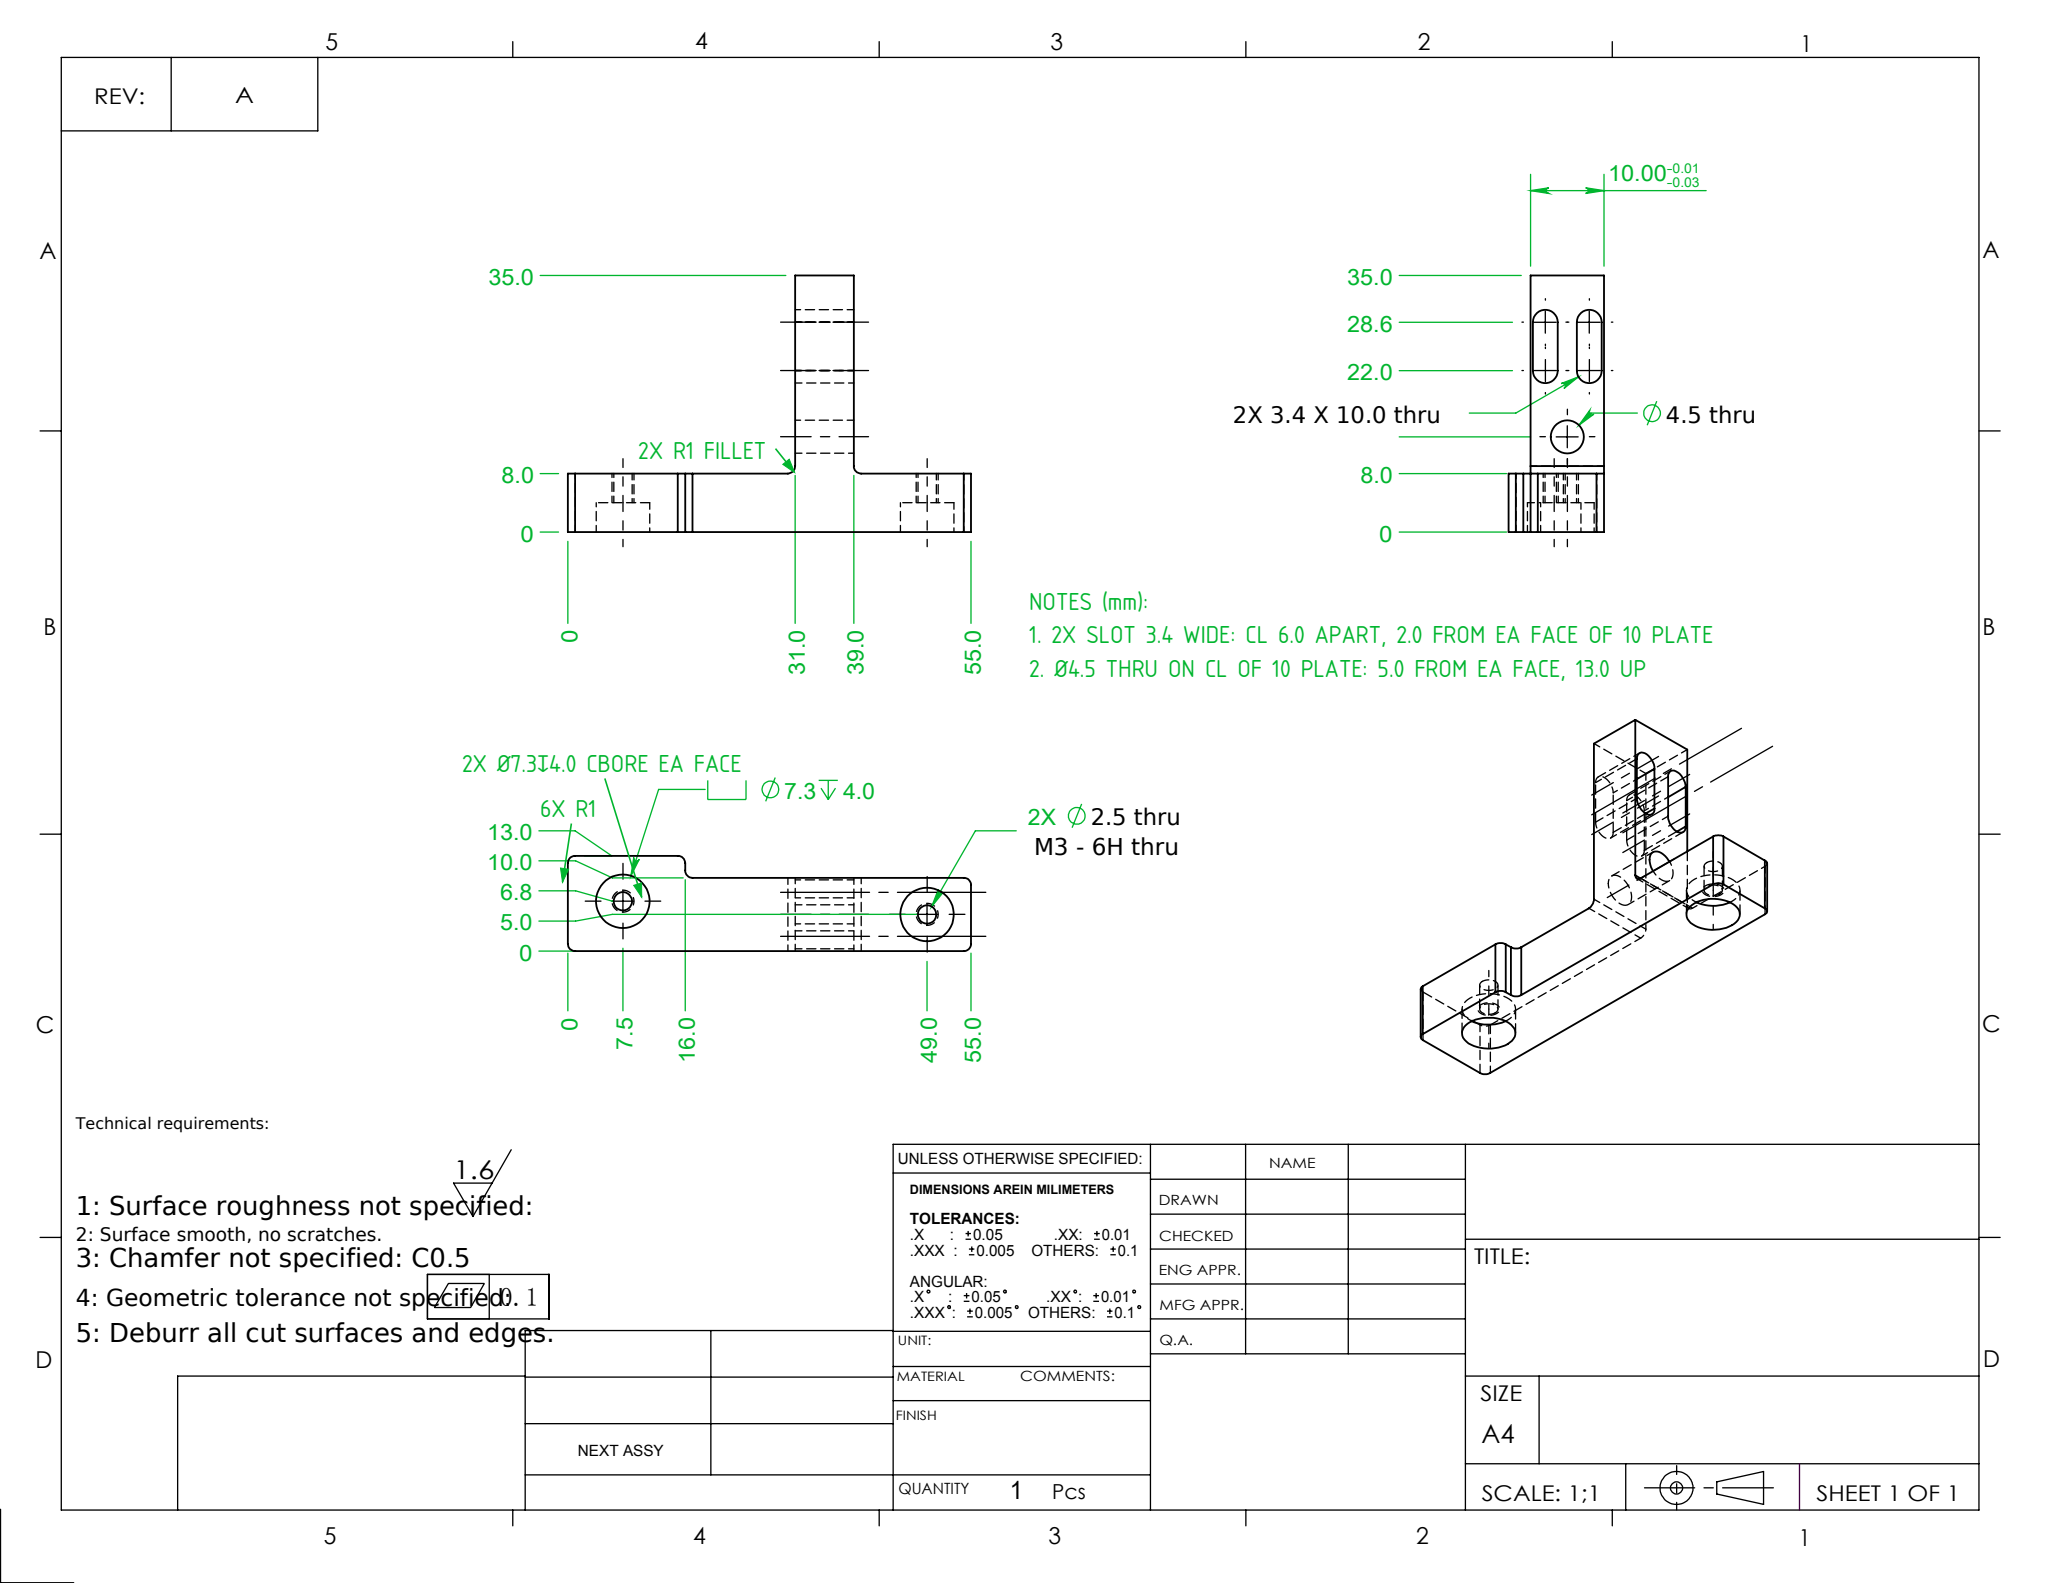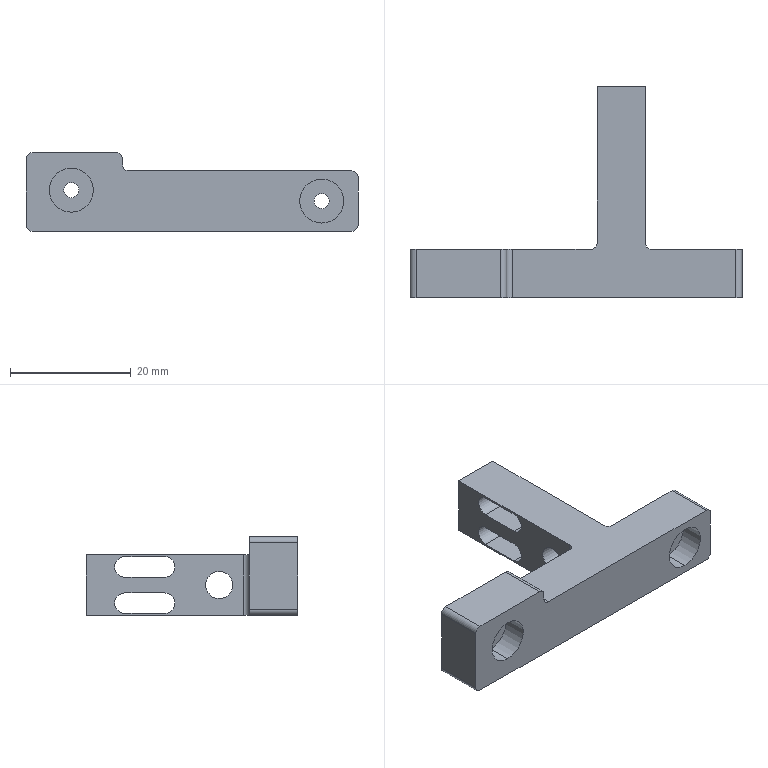Part | SolidWorks | mm | 1 solid | 40 faces | box 55 x 35 x 13 mm | volume 5936 mm3 | cylinder 22 | plane 18 | commonest cylinder face diameters 2 x8 2.5 x4 7.3 x4 3.4 x4 4.5 x2
Drawing notes:
2X SLOT 3.4 WIDE: CL 6.0 APART, 2.0 FROM EA FACE OF 10 PLATE | from the solid: 3.4 dia end cyls at z=2.0 & z=8.0 (y=22.02/28.62) in plate z=0..10; CL spacing 6.0, 2.0 to each face; slot overall 10.0 long in Y
Ø4.5 THRU ON CL OF 10 PLATE: 5.0 FROM EA FACE, 13.0 UP | from the solid: 4.5 dia cyl, axis X, pos y=13.0, z=5.0, len 8.0; plate faces z=0 & z=10 -> centred, 5.0 each side
2X R1 FILLET AT UPRIGHT TO BASE JUNCT, FULL 10 PLATE DEPTH | from the solid: 2.0 dia cyls, axis Z, at (x=30,y=9) and (x=40,y=9), len 10.0 = R1 fillets both sides of upright
6X R1 CORNER RND ON BASE PLATE OUTLINE (TOP VIEW), 8 HIGH | from the solid: 2.0 dia cyls, axis Y, len 8.0 at (x,z)=(1,1),(1,12),(15,12),(17,11),(54,1),(54,9)
2X Ø7.3 DP 4.0 C'BORE EA FACE; M3-6H THRU, Ø2.5 DP 4.0 EA FACE | from the solid: 7.3 dia y-axis cyl len 4.0 count 2 at x=7.5 & x=49.0; 2.5 dia y-axis cyl len 4.0 count 2 same locations; y planes 0/4/8